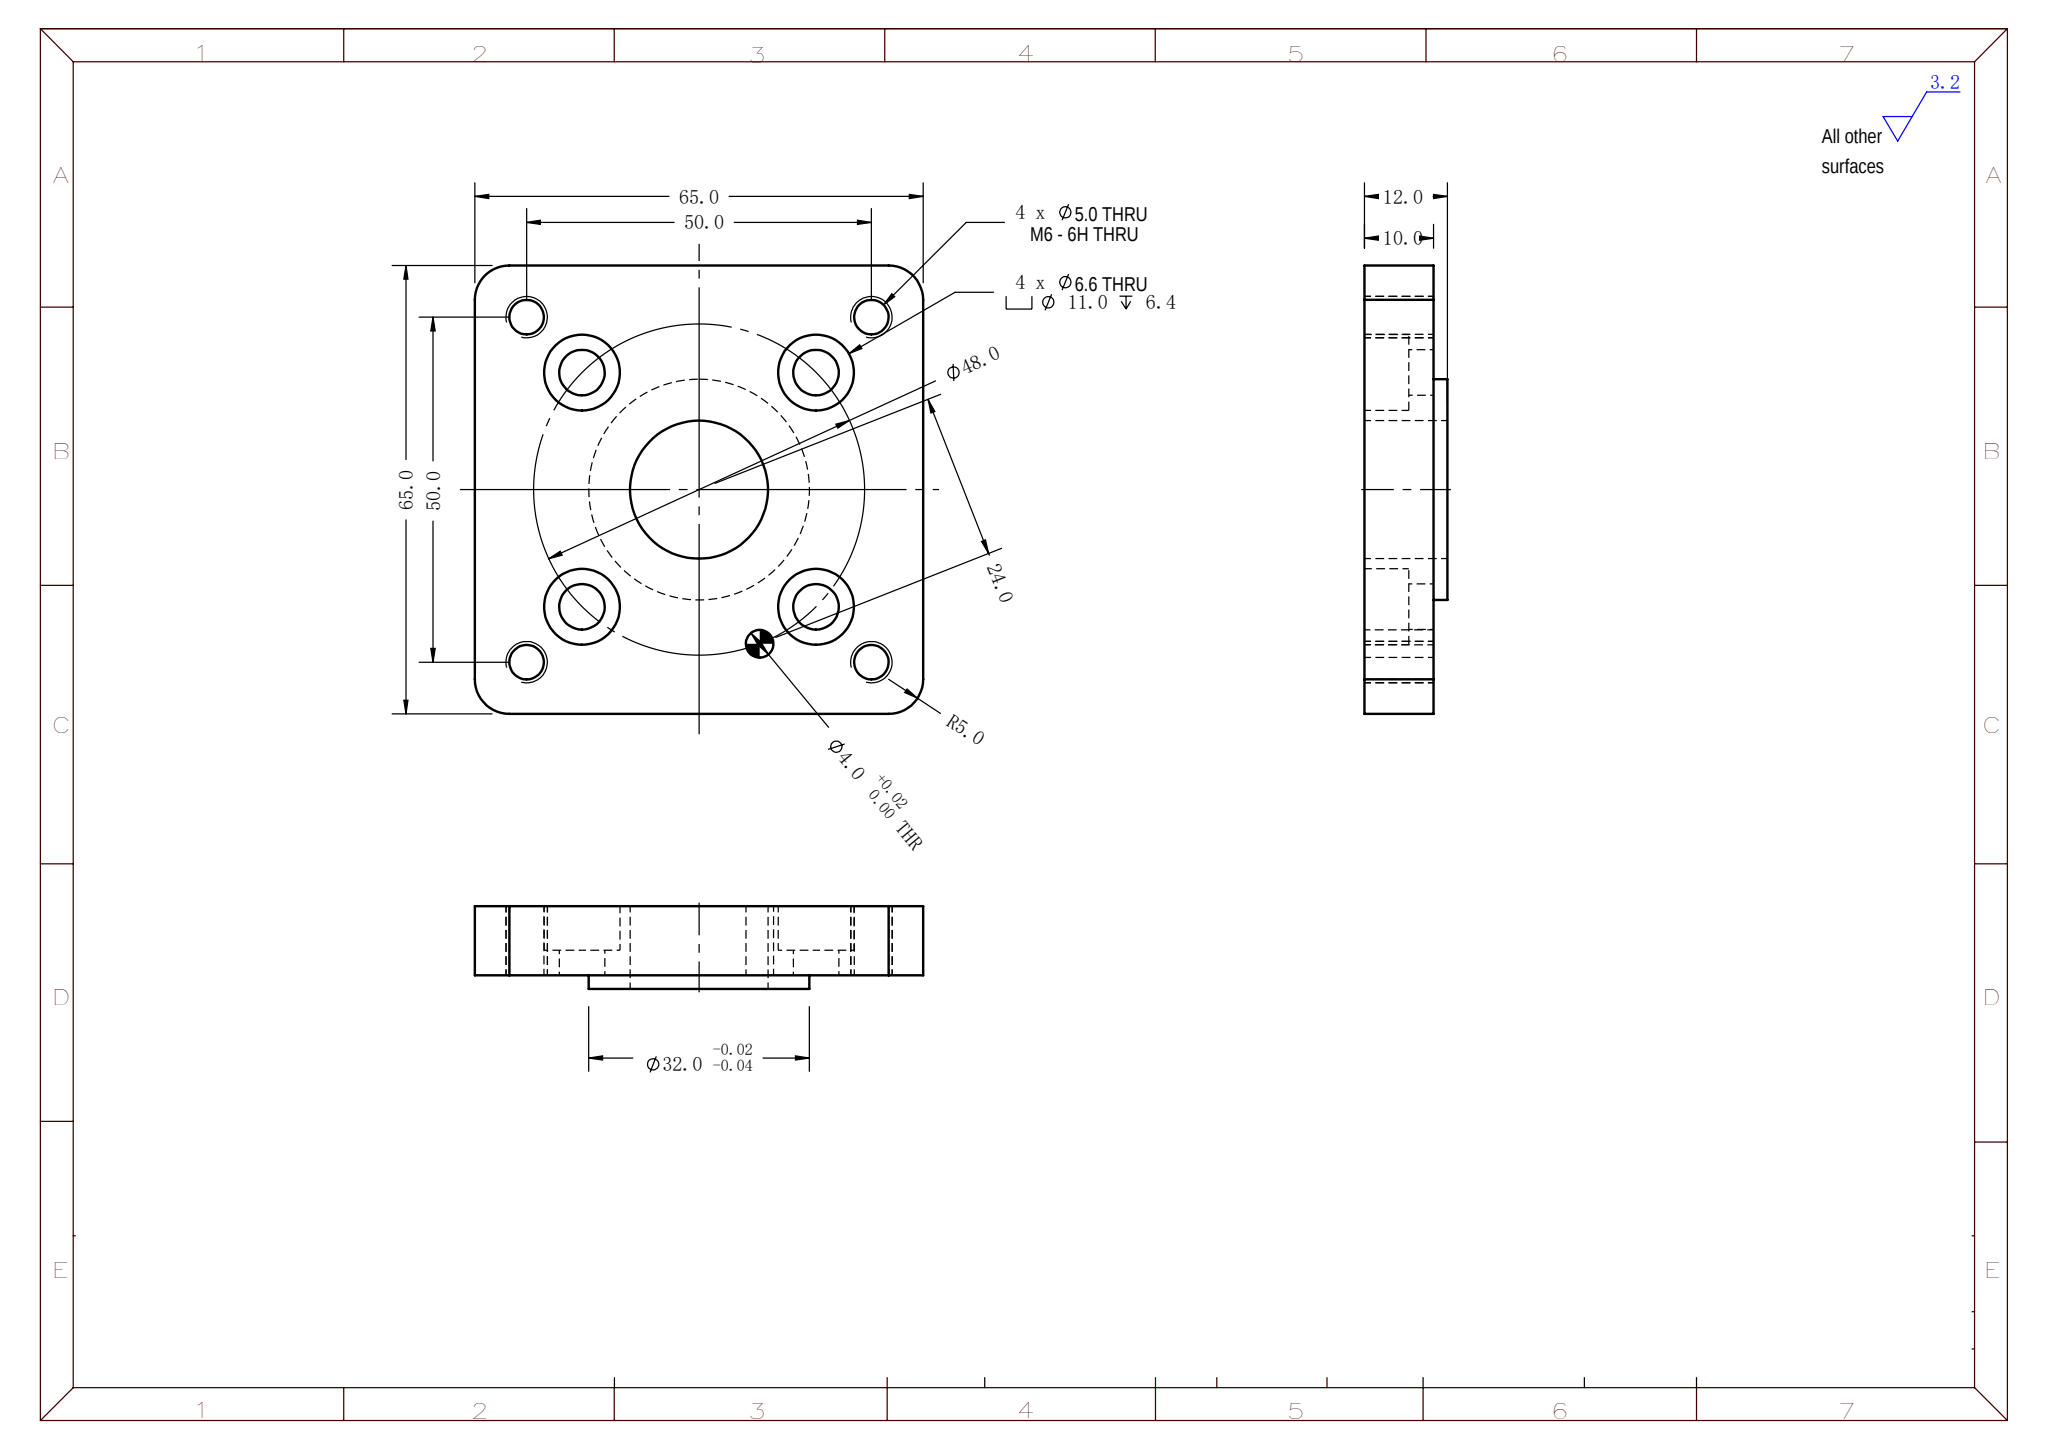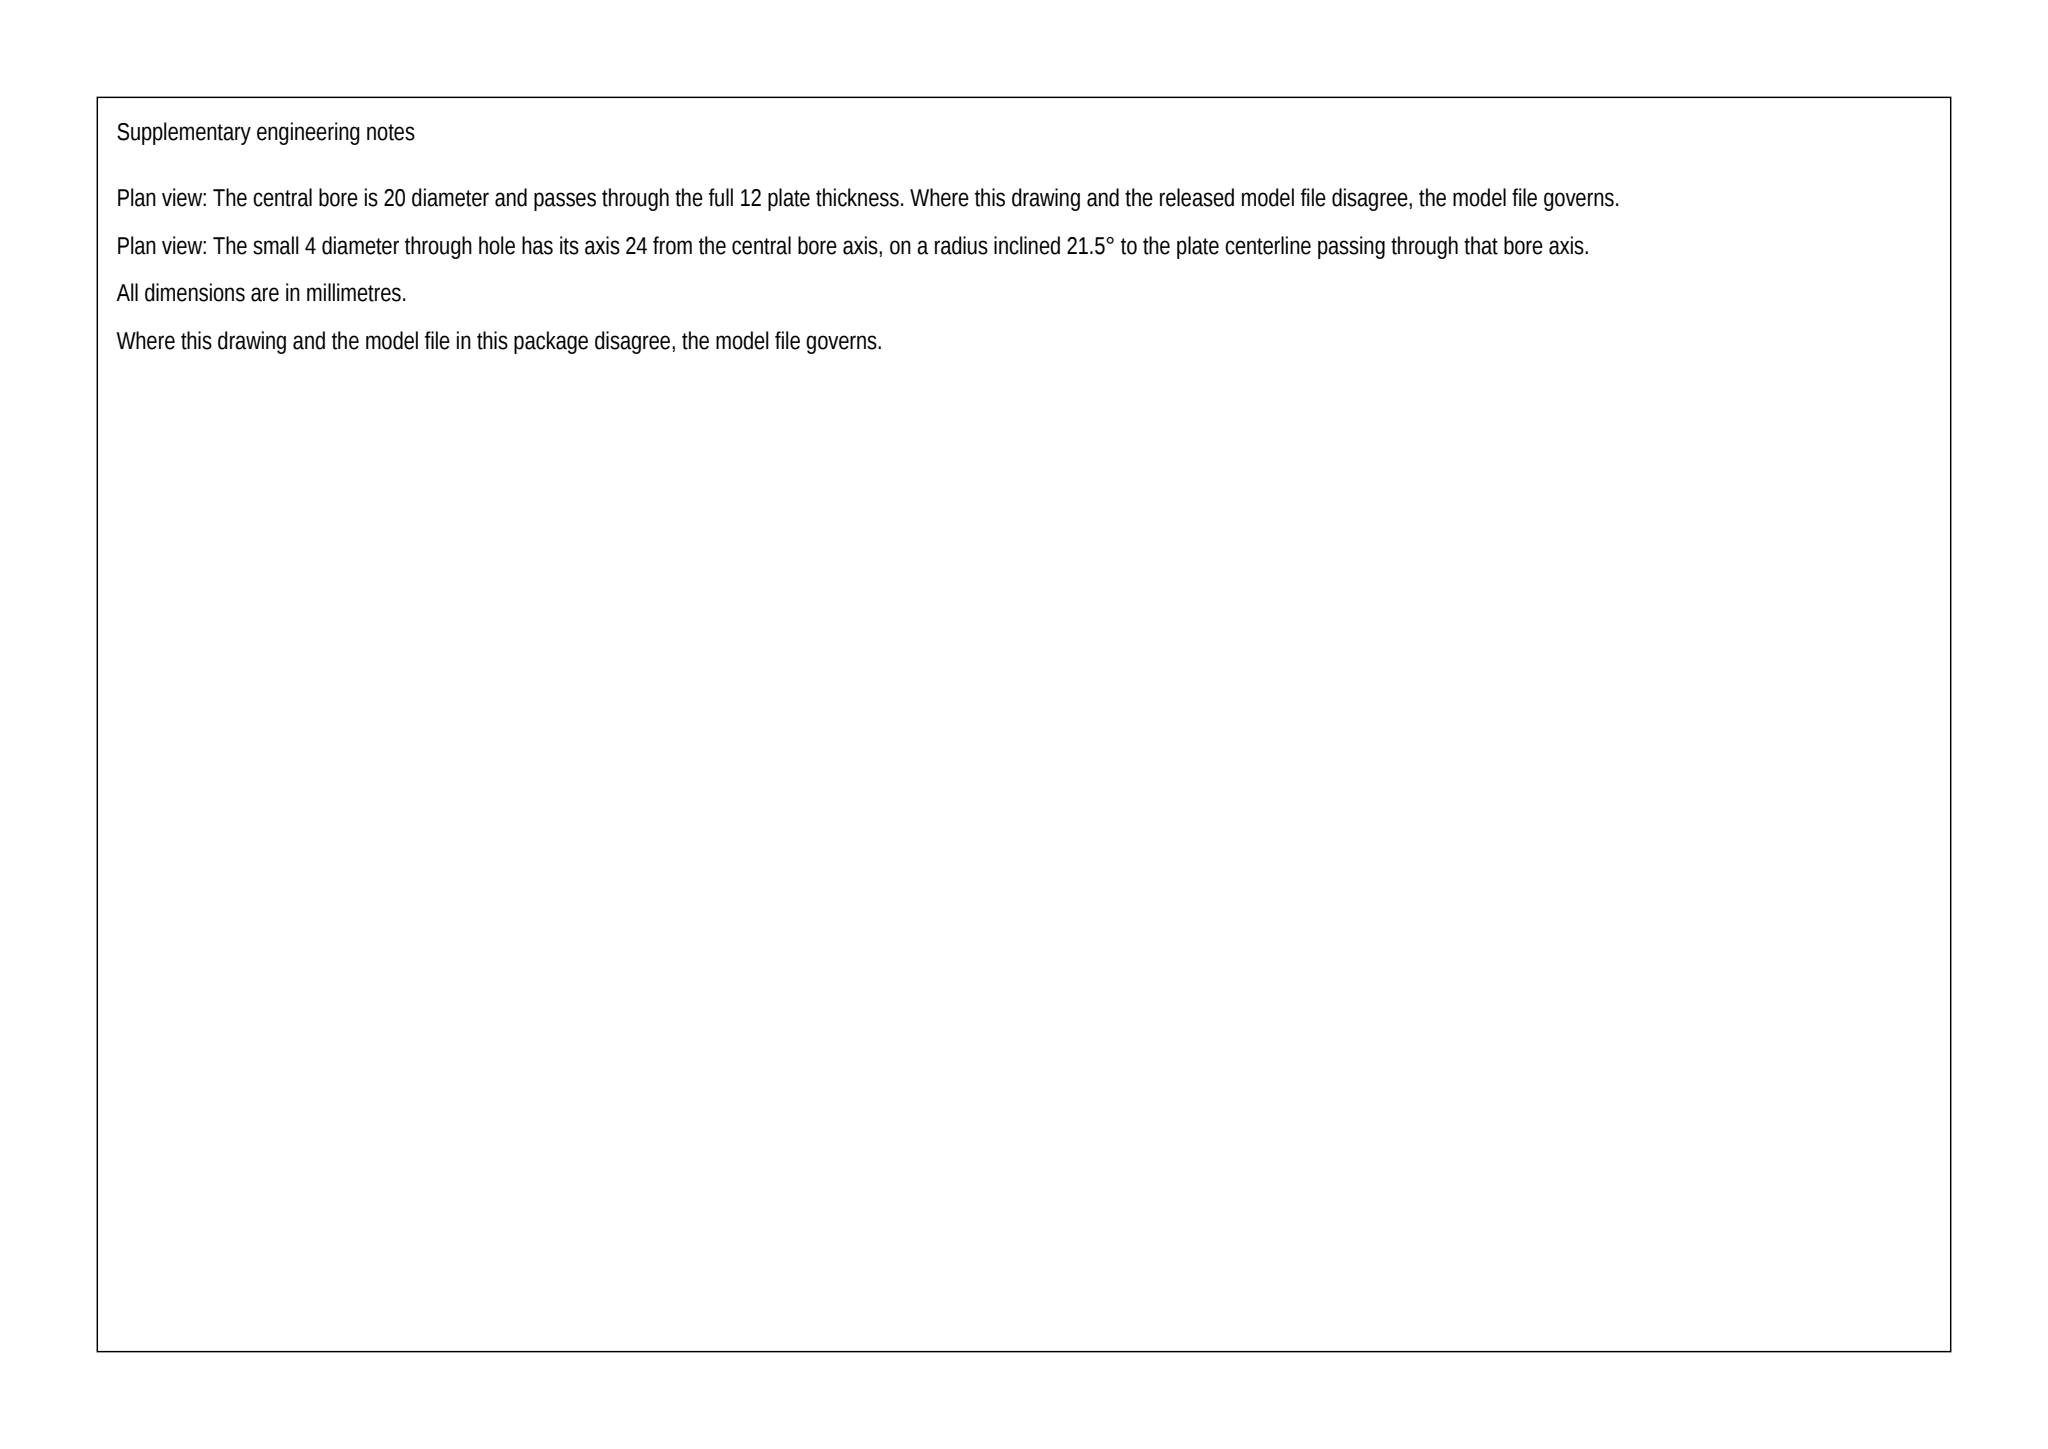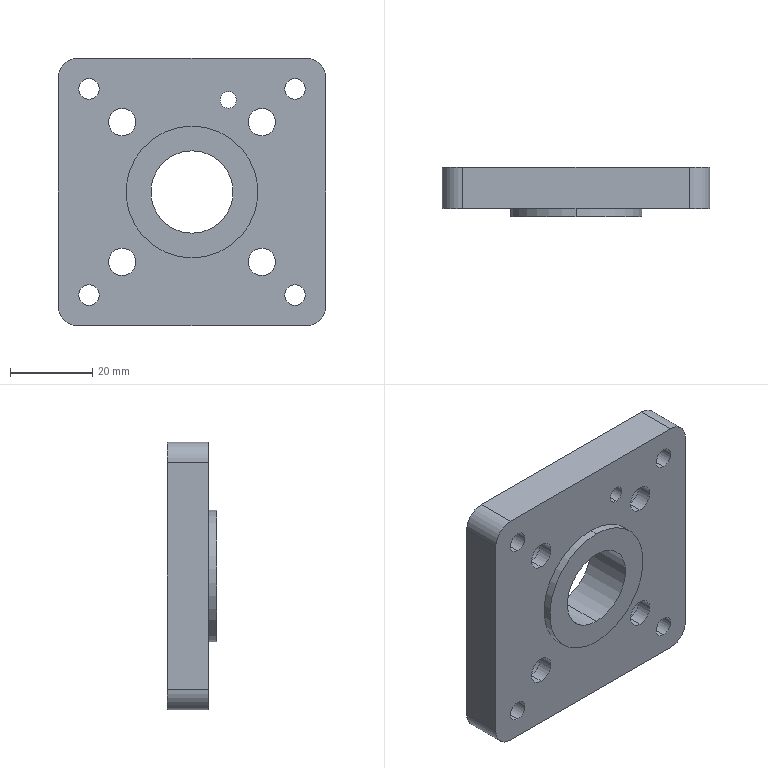Part | SolidWorks | mm | 1 solid | 45 faces | box 65 x 12 x 65 mm | volume 36037 mm3 | cylinder 34 | plane 11 | commonest cylinder face diameters 11 x8 6.6 x8 5 x8 10 x4 32 x2 20 x2 4 x2
build123d program:
from build123d import *

# Parameters (mm, degrees)
SKETCH1_W                                       = 65
SKETCH1_H                                       = 65
SKETCH1_R                                       = 10
SKETCH1_R_2                                     = 2
BOSS_EXTRUDE1_DEPTH                             = 6
M6_TAPPED_HOLE1_D                               = 5
FILLET1_R                                       = 5
SKETCH4_OUTSIDE_W                               = 85.54
SKETCH4_OUTSIDE_H                               = 85.54
SKETCH4_OUTSIDE_R                               = 16
CUT_EXTRUDE1_DEPTH                              = 2
M6_HEX_SOCKET_HEAD_CAP_SCREW_CBORE1_D           = 6.6
M6_HEX_SOCKET_HEAD_CAP_SCREW_CBORE1_CBORE_D     = 11
M6_HEX_SOCKET_HEAD_CAP_SCREW_CBORE1_CBORE_DEPTH = 6.4


with BuildPart() as part:
    # Sketch1 → Boss-Extrude1 (new, symmetric)
    with BuildSketch(Plane(origin=(0, 0, 0), x_dir=(1, 0, 0), z_dir=(0, 1, 0))):
        Rectangle(SKETCH1_W, SKETCH1_H)
        with Locations(Location((0, 0, 0), (0, 0, 270))):
            Circle(SKETCH1_R, mode=Mode.SUBTRACT)
        with Locations(Location((8.796, -22.33, 0), (0, 0, 270))):
            Circle(SKETCH1_R_2, mode=Mode.SUBTRACT)
    extrude(amount=BOSS_EXTRUDE1_DEPTH, both=True)

    # M6 Tapped Hole1 (through all)
    with Locations(Plane(origin=(0, 6, 0), x_dir=(1, 0, 0), z_dir=(0, 1, 0))):
        with Locations((25, 25), (-25, 25), (-25, -25), (25, -25)):
            Hole(M6_TAPPED_HOLE1_D / 2)

    # Fillet1
    fillet1_edges = [part.edges().sort_by_distance(p)[0] for p in [
        (-32.5, 0, -32.5),
        (32.5, 0, -32.5),
        (32.5, 0, 32.5),
        (-32.5, 0, 32.5),
    ]]
    fillet(fillet1_edges, radius=FILLET1_R)

    # Sketch4 outside → Cut-Extrude1 (cut)
    with BuildSketch(Plane.XZ.offset(6)):
        Rectangle(SKETCH4_OUTSIDE_W, SKETCH4_OUTSIDE_H)
        with Locations(Location((0, 0, 0), (0, 0, 270))):
            Circle(SKETCH4_OUTSIDE_R, mode=Mode.SUBTRACT)
    extrude(amount=-CUT_EXTRUDE1_DEPTH, mode=Mode.SUBTRACT)

    # M6 Hex Socket Head Cap Screw CBORE1 (through all)
    with Locations(Plane(origin=(0, 6, 0), x_dir=(1, 0, 0), z_dir=(0, 1, 0))):
        with Locations((16.971, 16.971), (-16.971, 16.971), (-16.971, -16.971), (16.971, -16.971)):
            CounterBoreHole(M6_HEX_SOCKET_HEAD_CAP_SCREW_CBORE1_D / 2, M6_HEX_SOCKET_HEAD_CAP_SCREW_CBORE1_CBORE_D / 2, M6_HEX_SOCKET_HEAD_CAP_SCREW_CBORE1_CBORE_DEPTH)


solid = part.part